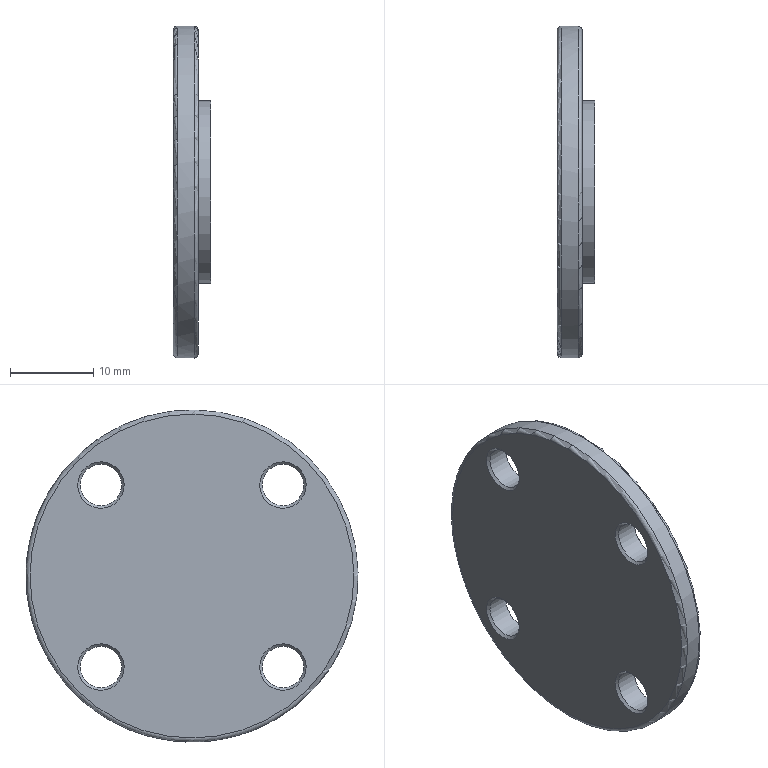Component | NX | UPPER_END_CAP_2 | 1 solid | 15 faces | box 4.5 x 40 x 40 mm | volume 4088 mm3 | cylinder 6 | cone 4 | plane 3 | torus 2 | commonest cylinder face diameters 5 x4 22 x1 40 x1
STEP:
#1=CARTESIAN_POINT('',(0.,0.,0.));
#2=DIRECTION('',(0.,0.,1.));
#3=DIRECTION('',(1.,0.,0.));
#4=AXIS2_PLACEMENT_3D('',#1,#2,#3);
#5=CARTESIAN_POINT('',(-135.,-29.778,26.278));
#6=VERTEX_POINT('',#5);
#7=CARTESIAN_POINT('',(-135.,-22.,18.5));
#8=DIRECTION('',(-1.,0.,0.));
#9=DIRECTION('',(0.,-0.7071,0.7071));
#10=AXIS2_PLACEMENT_3D('',#7,#8,#9);
#11=CIRCLE('',#10,11.);
#12=CARTESIAN_POINT('',(-135.,-22.,18.5));
#13=DIRECTION('',(1.,0.,0.));
#14=DIRECTION('',(0.,0.7071,-0.7071));
#15=AXIS2_PLACEMENT_3D('',#12,#13,#14);
#16=PLANE('',#15);
#17=CARTESIAN_POINT('',(-11.,-0.));
#18=CARTESIAN_POINT('',(-11.,19.053));
#19=CARTESIAN_POINT('',(5.5,9.526));
#20=CARTESIAN_POINT('',(22.,0.));
#21=CARTESIAN_POINT('',(5.5,-9.526));
#22=CARTESIAN_POINT('',(-11.,-19.053));
#23=CARTESIAN_POINT('',(-11.,-0.));
#24=(BOUNDED_CURVE()B_SPLINE_CURVE(2,(#17,#18,#19,#20,#21,#22,#23),.UNSPECIFIED.,.T.,.F.)B_SPLINE_CURVE_WITH_KNOTS((1,2,2,2,2,1),(-2.094,0.,2.094,4.189,6.283,8.378),.UNSPECIFIED.)CURVE()GEOMETRIC_REPRESENTATION_ITEM()RATIONAL_B_SPLINE_CURVE((1.,0.5,1.,0.5,1.,0.5,1.))REPRESENTATION_ITEM(''));
#25=(GEOMETRIC_REPRESENTATION_CONTEXT(2)PARAMETRIC_REPRESENTATION_CONTEXT()REPRESENTATION_CONTEXT('',''));
#26=DEFINITIONAL_REPRESENTATION('',(#24),#25);
#27=PCURVE('',#16,#26);
#28=CARTESIAN_POINT('',(-135.,-22.,18.5));
#29=DIRECTION('',(-1.,0.,0.));
#30=DIRECTION('',(0.,-0.7071,0.7071));
#31=AXIS2_PLACEMENT_3D('',#28,#29,#30);
#32=CYLINDRICAL_SURFACE('',#31,11.);
#33=CARTESIAN_POINT('',(0.,0.));
#34=DIRECTION('',(1.,0.));
#35=VECTOR('',#34,1.);
#36=LINE('',#33,#35);
#37=(GEOMETRIC_REPRESENTATION_CONTEXT(2)PARAMETRIC_REPRESENTATION_CONTEXT()REPRESENTATION_CONTEXT('',''));
#38=DEFINITIONAL_REPRESENTATION('',(#36),#37);
#39=PCURVE('',#32,#38);
#40=SURFACE_CURVE('',#11,(#27,#39),.PCURVE_S1.);
#41=EDGE_CURVE('',#6,#6,#40,.T.);
#42=ORIENTED_EDGE('',*,*,#41,.F.);
#43=EDGE_LOOP('',(#42));
#44=FACE_BOUND('',#43,.T.);
#45=ADVANCED_FACE('',(#44),#16,.T.);
#46=CARTESIAN_POINT('',(-136.5,-29.778,26.278));
#47=VERTEX_POINT('',#46);
#48=CARTESIAN_POINT('',(-136.5,-22.,18.5));
#49=DIRECTION('',(1.,0.,0.));
#50=DIRECTION('',(0.,-0.7071,0.7071));
#51=AXIS2_PLACEMENT_3D('',#48,#49,#50);
#52=CIRCLE('',#51,11.);
#53=CARTESIAN_POINT('',(6.283,1.5));
#54=DIRECTION('',(-1.,0.));
#55=VECTOR('',#54,1.);
#56=LINE('',#53,#55);
#57=(GEOMETRIC_REPRESENTATION_CONTEXT(2)PARAMETRIC_REPRESENTATION_CONTEXT()REPRESENTATION_CONTEXT('',''));
#58=DEFINITIONAL_REPRESENTATION('',(#56),#57);
#59=PCURVE('',#32,#58);
#60=CARTESIAN_POINT('',(-136.5,-22.,18.5));
#61=DIRECTION('',(1.,0.,0.));
#62=DIRECTION('',(0.,0.7071,-0.7071));
#63=AXIS2_PLACEMENT_3D('',#60,#61,#62);
#64=PLANE('',#63);
#65=CARTESIAN_POINT('',(0.,0.));
#66=DIRECTION('',(-1.,-0.));
#67=AXIS2_PLACEMENT_2D('',#65,#66);
#68=CIRCLE('',#67,11.);
#69=(GEOMETRIC_REPRESENTATION_CONTEXT(2)PARAMETRIC_REPRESENTATION_CONTEXT()REPRESENTATION_CONTEXT('',''));
#70=DEFINITIONAL_REPRESENTATION('',(#68),#69);
#71=PCURVE('',#64,#70);
#72=SURFACE_CURVE('',#52,(#59,#71),.PCURVE_S1.);
#73=EDGE_CURVE('',#47,#47,#72,.T.);
#74=ORIENTED_EDGE('',*,*,#73,.T.);
#75=CARTESIAN_POINT('',(-135.,-29.778,26.278));
#76=CARTESIAN_POINT('',(-136.5,-29.778,26.278));
#77=B_SPLINE_CURVE_WITH_KNOTS('',1,(#75,#76),.UNSPECIFIED.,.F.,.F.,(2,2),(0.,1.5),.PIECEWISE_BEZIER_KNOTS.);
#78=CARTESIAN_POINT('',(0.,0.));
#79=DIRECTION('',(0.,1.));
#80=VECTOR('',#79,1.);
#81=LINE('',#78,#80);
#82=(GEOMETRIC_REPRESENTATION_CONTEXT(2)PARAMETRIC_REPRESENTATION_CONTEXT()REPRESENTATION_CONTEXT('',''));
#83=DEFINITIONAL_REPRESENTATION('',(#81),#82);
#84=PCURVE('',#32,#83);
#85=CARTESIAN_POINT('',(6.283,0.));
#86=DIRECTION('',(0.,1.));
#87=VECTOR('',#86,1.);
#88=LINE('',#85,#87);
#89=(GEOMETRIC_REPRESENTATION_CONTEXT(2)PARAMETRIC_REPRESENTATION_CONTEXT()REPRESENTATION_CONTEXT('',''));
#90=DEFINITIONAL_REPRESENTATION('',(#88),#89);
#91=PCURVE('',#32,#90);
#92=SEAM_CURVE('',#77,(#84,#91),.PCURVE_S1.);
#93=EDGE_CURVE('',#6,#47,#92,.T.);
#94=ORIENTED_EDGE('',*,*,#93,.F.);
#95=ORIENTED_EDGE('',*,*,#41,.T.);
#96=ORIENTED_EDGE('',*,*,#93,.T.);
#97=EDGE_LOOP('',(#74,#94,#95,#96));
#98=FACE_BOUND('',#97,.T.);
#99=ADVANCED_FACE('',(#98),#32,.T.);
#100=CARTESIAN_POINT('',(-139.5,-13.02,9.52));
#101=VERTEX_POINT('',#100);
#102=CARTESIAN_POINT('',(-139.5,-11.04,7.54));
#103=DIRECTION('',(1.,0.,0.));
#104=DIRECTION('',(0.,-0.7071,0.7071));
#105=AXIS2_PLACEMENT_3D('',#102,#103,#104);
#106=CIRCLE('',#105,2.8);
#107=CARTESIAN_POINT('',(-139.5,-22.,18.5));
#108=DIRECTION('',(-1.,0.,0.));
#109=DIRECTION('',(0.,-0.7071,0.7071));
#110=AXIS2_PLACEMENT_3D('',#107,#108,#109);
#111=PLANE('',#110);
#112=CARTESIAN_POINT('',(-12.7,0.));
#113=CARTESIAN_POINT('',(-12.7,-4.85));
#114=CARTESIAN_POINT('',(-16.9,-2.425));
#115=CARTESIAN_POINT('',(-21.1,0.));
#116=CARTESIAN_POINT('',(-16.9,2.425));
#117=CARTESIAN_POINT('',(-12.7,4.85));
#118=CARTESIAN_POINT('',(-12.7,0.));
#119=(BOUNDED_CURVE()B_SPLINE_CURVE(2,(#112,#113,#114,#115,#116,#117,#118),.UNSPECIFIED.,.T.,.F.)B_SPLINE_CURVE_WITH_KNOTS((1,2,2,2,2,1),(-2.094,0.,2.094,4.189,6.283,8.378),.UNSPECIFIED.)CURVE()GEOMETRIC_REPRESENTATION_ITEM()RATIONAL_B_SPLINE_CURVE((1.,0.5,1.,0.5,1.,0.5,1.))REPRESENTATION_ITEM(''));
#120=(GEOMETRIC_REPRESENTATION_CONTEXT(2)PARAMETRIC_REPRESENTATION_CONTEXT()REPRESENTATION_CONTEXT('',''));
#121=DEFINITIONAL_REPRESENTATION('',(#119),#120);
#122=PCURVE('',#111,#121);
#123=CARTESIAN_POINT('',(-139.2,-11.04,7.54));
#124=DIRECTION('',(-1.,0.,0.));
#125=DIRECTION('',(0.,-0.7071,0.7071));
#126=AXIS2_PLACEMENT_3D('',#123,#124,#125);
#127=CONICAL_SURFACE('',#126,2.5,0.7854);
#128=CARTESIAN_POINT('',(6.283,0.3));
#129=DIRECTION('',(-1.,0.));
#130=VECTOR('',#129,1.);
#131=LINE('',#128,#130);
#132=(GEOMETRIC_REPRESENTATION_CONTEXT(2)PARAMETRIC_REPRESENTATION_CONTEXT()REPRESENTATION_CONTEXT('',''));
#133=DEFINITIONAL_REPRESENTATION('',(#131),#132);
#134=PCURVE('',#127,#133);
#135=SURFACE_CURVE('',#106,(#122,#134),.PCURVE_S1.);
#136=EDGE_CURVE('',#101,#101,#135,.T.);
#137=ORIENTED_EDGE('',*,*,#136,.T.);
#138=EDGE_LOOP('',(#137));
#139=FACE_BOUND('',#138,.T.);
#140=CARTESIAN_POINT('',(-139.5,-34.94,9.52));
#141=VERTEX_POINT('',#140);
#142=CARTESIAN_POINT('',(-139.5,-32.96,7.54));
#143=DIRECTION('',(1.,0.,0.));
#144=DIRECTION('',(0.,-0.7071,0.7071));
#145=AXIS2_PLACEMENT_3D('',#142,#143,#144);
#146=CIRCLE('',#145,2.8);
#147=CARTESIAN_POINT('',(2.8,-15.5));
#148=CARTESIAN_POINT('',(2.8,-20.35));
#149=CARTESIAN_POINT('',(-1.4,-17.925));
#150=CARTESIAN_POINT('',(-5.6,-15.5));
#151=CARTESIAN_POINT('',(-1.4,-13.075));
#152=CARTESIAN_POINT('',(2.8,-10.65));
#153=CARTESIAN_POINT('',(2.8,-15.5));
#154=(BOUNDED_CURVE()B_SPLINE_CURVE(2,(#147,#148,#149,#150,#151,#152,#153),.UNSPECIFIED.,.T.,.F.)B_SPLINE_CURVE_WITH_KNOTS((1,2,2,2,2,1),(-2.094,0.,2.094,4.189,6.283,8.378),.UNSPECIFIED.)CURVE()GEOMETRIC_REPRESENTATION_ITEM()RATIONAL_B_SPLINE_CURVE((1.,0.5,1.,0.5,1.,0.5,1.))REPRESENTATION_ITEM(''));
#155=(GEOMETRIC_REPRESENTATION_CONTEXT(2)PARAMETRIC_REPRESENTATION_CONTEXT()REPRESENTATION_CONTEXT('',''));
#156=DEFINITIONAL_REPRESENTATION('',(#154),#155);
#157=PCURVE('',#111,#156);
#158=CARTESIAN_POINT('',(-139.2,-32.96,7.54));
#159=DIRECTION('',(-1.,0.,0.));
#160=DIRECTION('',(0.,-0.7071,0.7071));
#161=AXIS2_PLACEMENT_3D('',#158,#159,#160);
#162=CONICAL_SURFACE('',#161,2.5,0.7854);
#163=CARTESIAN_POINT('',(6.283,0.3));
#164=DIRECTION('',(-1.,0.));
#165=VECTOR('',#164,1.);
#166=LINE('',#163,#165);
#167=(GEOMETRIC_REPRESENTATION_CONTEXT(2)PARAMETRIC_REPRESENTATION_CONTEXT()REPRESENTATION_CONTEXT('',''));
#168=DEFINITIONAL_REPRESENTATION('',(#166),#167);
#169=PCURVE('',#162,#168);
#170=SURFACE_CURVE('',#146,(#157,#169),.PCURVE_S1.);
#171=EDGE_CURVE('',#141,#141,#170,.T.);
#172=ORIENTED_EDGE('',*,*,#171,.T.);
#173=EDGE_LOOP('',(#172));
#174=FACE_BOUND('',#173,.T.);
#175=CARTESIAN_POINT('',(-139.5,-13.02,31.44));
#176=VERTEX_POINT('',#175);
#177=CARTESIAN_POINT('',(-139.5,-11.04,29.46));
#178=DIRECTION('',(1.,0.,0.));
#179=DIRECTION('',(0.,-0.7071,0.7071));
#180=AXIS2_PLACEMENT_3D('',#177,#178,#179);
#181=CIRCLE('',#180,2.8);
#182=CARTESIAN_POINT('',(2.8,15.5));
#183=CARTESIAN_POINT('',(2.8,10.65));
#184=CARTESIAN_POINT('',(-1.4,13.075));
#185=CARTESIAN_POINT('',(-5.6,15.5));
#186=CARTESIAN_POINT('',(-1.4,17.925));
#187=CARTESIAN_POINT('',(2.8,20.35));
#188=CARTESIAN_POINT('',(2.8,15.5));
#189=(BOUNDED_CURVE()B_SPLINE_CURVE(2,(#182,#183,#184,#185,#186,#187,#188),.UNSPECIFIED.,.T.,.F.)B_SPLINE_CURVE_WITH_KNOTS((1,2,2,2,2,1),(-2.094,0.,2.094,4.189,6.283,8.378),.UNSPECIFIED.)CURVE()GEOMETRIC_REPRESENTATION_ITEM()RATIONAL_B_SPLINE_CURVE((1.,0.5,1.,0.5,1.,0.5,1.))REPRESENTATION_ITEM(''));
#190=(GEOMETRIC_REPRESENTATION_CONTEXT(2)PARAMETRIC_REPRESENTATION_CONTEXT()REPRESENTATION_CONTEXT('',''));
#191=DEFINITIONAL_REPRESENTATION('',(#189),#190);
#192=PCURVE('',#111,#191);
#193=CARTESIAN_POINT('',(-139.2,-11.04,29.46));
#194=DIRECTION('',(-1.,0.,0.));
#195=DIRECTION('',(0.,-0.7071,0.7071));
#196=AXIS2_PLACEMENT_3D('',#193,#194,#195);
#197=CONICAL_SURFACE('',#196,2.5,0.7854);
#198=CARTESIAN_POINT('',(6.283,0.3));
#199=DIRECTION('',(-1.,0.));
#200=VECTOR('',#199,1.);
#201=LINE('',#198,#200);
#202=(GEOMETRIC_REPRESENTATION_CONTEXT(2)PARAMETRIC_REPRESENTATION_CONTEXT()REPRESENTATION_CONTEXT('',''));
#203=DEFINITIONAL_REPRESENTATION('',(#201),#202);
#204=PCURVE('',#197,#203);
#205=SURFACE_CURVE('',#181,(#192,#204),.PCURVE_S1.);
#206=EDGE_CURVE('',#176,#176,#205,.T.);
#207=ORIENTED_EDGE('',*,*,#206,.T.);
#208=EDGE_LOOP('',(#207));
#209=FACE_BOUND('',#208,.T.);
#210=CARTESIAN_POINT('',(-139.5,-34.94,31.44));
#211=VERTEX_POINT('',#210);
#212=CARTESIAN_POINT('',(-139.5,-32.96,29.46));
#213=DIRECTION('',(1.,0.,0.));
#214=DIRECTION('',(0.,-0.7071,0.7071));
#215=AXIS2_PLACEMENT_3D('',#212,#213,#214);
#216=CIRCLE('',#215,2.8);
#217=CARTESIAN_POINT('',(18.3,0.));
#218=CARTESIAN_POINT('',(18.3,-4.85));
#219=CARTESIAN_POINT('',(14.1,-2.425));
#220=CARTESIAN_POINT('',(9.9,0.));
#221=CARTESIAN_POINT('',(14.1,2.425));
#222=CARTESIAN_POINT('',(18.3,4.85));
#223=CARTESIAN_POINT('',(18.3,0.));
#224=(BOUNDED_CURVE()B_SPLINE_CURVE(2,(#217,#218,#219,#220,#221,#222,#223),.UNSPECIFIED.,.T.,.F.)B_SPLINE_CURVE_WITH_KNOTS((1,2,2,2,2,1),(-2.094,0.,2.094,4.189,6.283,8.378),.UNSPECIFIED.)CURVE()GEOMETRIC_REPRESENTATION_ITEM()RATIONAL_B_SPLINE_CURVE((1.,0.5,1.,0.5,1.,0.5,1.))REPRESENTATION_ITEM(''));
#225=(GEOMETRIC_REPRESENTATION_CONTEXT(2)PARAMETRIC_REPRESENTATION_CONTEXT()REPRESENTATION_CONTEXT('',''));
#226=DEFINITIONAL_REPRESENTATION('',(#224),#225);
#227=PCURVE('',#111,#226);
#228=CARTESIAN_POINT('',(-139.2,-32.96,29.46));
#229=DIRECTION('',(-1.,0.,0.));
#230=DIRECTION('',(0.,-0.7071,0.7071));
#231=AXIS2_PLACEMENT_3D('',#228,#229,#230);
#232=CONICAL_SURFACE('',#231,2.5,0.7854);
#233=CARTESIAN_POINT('',(6.283,0.3));
#234=DIRECTION('',(-1.,0.));
#235=VECTOR('',#234,1.);
#236=LINE('',#233,#235);
#237=(GEOMETRIC_REPRESENTATION_CONTEXT(2)PARAMETRIC_REPRESENTATION_CONTEXT()REPRESENTATION_CONTEXT('',''));
#238=DEFINITIONAL_REPRESENTATION('',(#236),#237);
#239=PCURVE('',#232,#238);
#240=SURFACE_CURVE('',#216,(#227,#239),.PCURVE_S1.);
#241=EDGE_CURVE('',#211,#211,#240,.T.);
#242=ORIENTED_EDGE('',*,*,#241,.T.);
#243=EDGE_LOOP('',(#242));
#244=FACE_BOUND('',#243,.T.);
#245=CARTESIAN_POINT('',(-139.5,-35.789,32.289));
#246=VERTEX_POINT('',#245);
#247=CARTESIAN_POINT('',(-139.5,-22.,18.5));
#248=DIRECTION('',(-1.,0.,0.));
#249=DIRECTION('',(0.,-0.7071,0.7071));
#250=AXIS2_PLACEMENT_3D('',#247,#248,#249);
#251=CIRCLE('',#250,19.5);
#252=CARTESIAN_POINT('',(0.,0.));
#253=DIRECTION('',(1.,0.));
#254=AXIS2_PLACEMENT_2D('',#252,#253);
#255=CIRCLE('',#254,19.5);
#256=(GEOMETRIC_REPRESENTATION_CONTEXT(2)PARAMETRIC_REPRESENTATION_CONTEXT()REPRESENTATION_CONTEXT('',''));
#257=DEFINITIONAL_REPRESENTATION('',(#255),#256);
#258=PCURVE('',#111,#257);
#259=CARTESIAN_POINT('',(-139.,-22.,18.5));
#260=DIRECTION('',(-1.,0.,0.));
#261=DIRECTION('',(0.,-0.7071,0.7071));
#262=AXIS2_PLACEMENT_3D('',#259,#260,#261);
#263=TOROIDAL_SURFACE('',#262,19.5,0.5);
#264=CARTESIAN_POINT('',(0.,7.854));
#265=DIRECTION('',(1.,0.));
#266=VECTOR('',#265,1.);
#267=LINE('',#264,#266);
#268=(GEOMETRIC_REPRESENTATION_CONTEXT(2)PARAMETRIC_REPRESENTATION_CONTEXT()REPRESENTATION_CONTEXT('',''));
#269=DEFINITIONAL_REPRESENTATION('',(#267),#268);
#270=PCURVE('',#263,#269);
#271=SURFACE_CURVE('',#251,(#258,#270),.PCURVE_S1.);
#272=EDGE_CURVE('',#246,#246,#271,.T.);
#273=ORIENTED_EDGE('',*,*,#272,.T.);
#274=EDGE_LOOP('',(#273));
#275=FACE_BOUND('',#274,.T.);
#276=ADVANCED_FACE('',(#139,#174,#209,#244,#275),#111,.T.);
#277=CARTESIAN_POINT('',(-136.5,-31.192,27.692));
#278=VERTEX_POINT('',#277);
#279=CARTESIAN_POINT('',(-136.5,-34.728,31.228));
#280=VERTEX_POINT('',#279);
#281=CARTESIAN_POINT('',(-136.5,-32.96,29.46));
#282=DIRECTION('',(1.,0.,0.));
#283=DIRECTION('',(0.,0.7071,-0.7071));
#284=AXIS2_PLACEMENT_3D('',#281,#282,#283);
#285=CIRCLE('',#284,2.5);
#286=CARTESIAN_POINT('',(-15.5,0.));
#287=DIRECTION('',(1.,0.));
#288=AXIS2_PLACEMENT_2D('',#286,#287);
#289=CIRCLE('',#288,2.5);
#290=(GEOMETRIC_REPRESENTATION_CONTEXT(2)PARAMETRIC_REPRESENTATION_CONTEXT()REPRESENTATION_CONTEXT('',''));
#291=DEFINITIONAL_REPRESENTATION('',(#289),#290);
#292=PCURVE('',#64,#291);
#293=CARTESIAN_POINT('',(-119.5,-32.96,29.46));
#294=DIRECTION('',(-1.,0.,0.));
#295=DIRECTION('',(0.,-0.7071,0.7071));
#296=AXIS2_PLACEMENT_3D('',#293,#294,#295);
#297=CYLINDRICAL_SURFACE('',#296,2.5);
#298=CARTESIAN_POINT('',(3.142,17.));
#299=DIRECTION('',(-1.,0.));
#300=VECTOR('',#299,1.);
#301=LINE('',#298,#300);
#302=(GEOMETRIC_REPRESENTATION_CONTEXT(2)PARAMETRIC_REPRESENTATION_CONTEXT()REPRESENTATION_CONTEXT('',''));
#303=DEFINITIONAL_REPRESENTATION('',(#301),#302);
#304=PCURVE('',#297,#303);
#305=SURFACE_CURVE('',#285,(#292,#304),.PCURVE_S1.);
#306=EDGE_CURVE('',#278,#280,#305,.T.);
#307=ORIENTED_EDGE('',*,*,#306,.F.);
#308=CARTESIAN_POINT('',(-136.5,-32.96,29.46));
#309=DIRECTION('',(1.,0.,0.));
#310=DIRECTION('',(0.,0.7071,-0.7071));
#311=AXIS2_PLACEMENT_3D('',#308,#309,#310);
#312=CIRCLE('',#311,2.5);
#313=CARTESIAN_POINT('',(-15.5,0.));
#314=DIRECTION('',(1.,0.));
#315=AXIS2_PLACEMENT_2D('',#313,#314);
#316=CIRCLE('',#315,2.5);
#317=(GEOMETRIC_REPRESENTATION_CONTEXT(2)PARAMETRIC_REPRESENTATION_CONTEXT()REPRESENTATION_CONTEXT('',''));
#318=DEFINITIONAL_REPRESENTATION('',(#316),#317);
#319=PCURVE('',#64,#318);
#320=CARTESIAN_POINT('',(9.425,17.));
#321=DIRECTION('',(-1.,0.));
#322=VECTOR('',#321,1.);
#323=LINE('',#320,#322);
#324=(GEOMETRIC_REPRESENTATION_CONTEXT(2)PARAMETRIC_REPRESENTATION_CONTEXT()REPRESENTATION_CONTEXT('',''));
#325=DEFINITIONAL_REPRESENTATION('',(#323),#324);
#326=PCURVE('',#297,#325);
#327=SURFACE_CURVE('',#312,(#319,#326),.PCURVE_S1.);
#328=EDGE_CURVE('',#280,#278,#327,.T.);
#329=ORIENTED_EDGE('',*,*,#328,.F.);
#330=EDGE_LOOP('',(#307,#329));
#331=FACE_BOUND('',#330,.T.);
#332=CARTESIAN_POINT('',(-136.5,-9.272,27.692));
#333=VERTEX_POINT('',#332);
#334=CARTESIAN_POINT('',(-136.5,-12.808,31.228));
#335=VERTEX_POINT('',#334);
#336=CARTESIAN_POINT('',(-136.5,-11.04,29.46));
#337=DIRECTION('',(1.,0.,0.));
#338=DIRECTION('',(0.,0.7071,-0.7071));
#339=AXIS2_PLACEMENT_3D('',#336,#337,#338);
#340=CIRCLE('',#339,2.5);
#341=CARTESIAN_POINT('',(-0.,15.5));
#342=DIRECTION('',(1.,0.));
#343=AXIS2_PLACEMENT_2D('',#341,#342);
#344=CIRCLE('',#343,2.5);
#345=(GEOMETRIC_REPRESENTATION_CONTEXT(2)PARAMETRIC_REPRESENTATION_CONTEXT()REPRESENTATION_CONTEXT('',''));
#346=DEFINITIONAL_REPRESENTATION('',(#344),#345);
#347=PCURVE('',#64,#346);
#348=CARTESIAN_POINT('',(-119.5,-11.04,29.46));
#349=DIRECTION('',(-1.,0.,0.));
#350=DIRECTION('',(0.,-0.7071,0.7071));
#351=AXIS2_PLACEMENT_3D('',#348,#349,#350);
#352=CYLINDRICAL_SURFACE('',#351,2.5);
#353=CARTESIAN_POINT('',(3.142,17.));
#354=DIRECTION('',(-1.,0.));
#355=VECTOR('',#354,1.);
#356=LINE('',#353,#355);
#357=(GEOMETRIC_REPRESENTATION_CONTEXT(2)PARAMETRIC_REPRESENTATION_CONTEXT()REPRESENTATION_CONTEXT('',''));
#358=DEFINITIONAL_REPRESENTATION('',(#356),#357);
#359=PCURVE('',#352,#358);
#360=SURFACE_CURVE('',#340,(#347,#359),.PCURVE_S1.);
#361=EDGE_CURVE('',#333,#335,#360,.T.);
#362=ORIENTED_EDGE('',*,*,#361,.F.);
#363=CARTESIAN_POINT('',(-136.5,-11.04,29.46));
#364=DIRECTION('',(1.,0.,0.));
#365=DIRECTION('',(0.,0.7071,-0.7071));
#366=AXIS2_PLACEMENT_3D('',#363,#364,#365);
#367=CIRCLE('',#366,2.5);
#368=CARTESIAN_POINT('',(-0.,15.5));
#369=DIRECTION('',(1.,0.));
#370=AXIS2_PLACEMENT_2D('',#368,#369);
#371=CIRCLE('',#370,2.5);
#372=(GEOMETRIC_REPRESENTATION_CONTEXT(2)PARAMETRIC_REPRESENTATION_CONTEXT()REPRESENTATION_CONTEXT('',''));
#373=DEFINITIONAL_REPRESENTATION('',(#371),#372);
#374=PCURVE('',#64,#373);
#375=CARTESIAN_POINT('',(9.425,17.));
#376=DIRECTION('',(-1.,0.));
#377=VECTOR('',#376,1.);
#378=LINE('',#375,#377);
#379=(GEOMETRIC_REPRESENTATION_CONTEXT(2)PARAMETRIC_REPRESENTATION_CONTEXT()REPRESENTATION_CONTEXT('',''));
#380=DEFINITIONAL_REPRESENTATION('',(#378),#379);
#381=PCURVE('',#352,#380);
#382=SURFACE_CURVE('',#367,(#374,#381),.PCURVE_S1.);
#383=EDGE_CURVE('',#335,#333,#382,.T.);
#384=ORIENTED_EDGE('',*,*,#383,.F.);
#385=EDGE_LOOP('',(#362,#384));
#386=FACE_BOUND('',#385,.T.);
#387=CARTESIAN_POINT('',(-136.5,-31.192,5.772));
#388=VERTEX_POINT('',#387);
#389=CARTESIAN_POINT('',(-136.5,-34.728,9.308));
#390=VERTEX_POINT('',#389);
#391=CARTESIAN_POINT('',(-136.5,-32.96,7.54));
#392=DIRECTION('',(1.,0.,0.));
#393=DIRECTION('',(0.,0.7071,-0.7071));
#394=AXIS2_PLACEMENT_3D('',#391,#392,#393);
#395=CIRCLE('',#394,2.5);
#396=CARTESIAN_POINT('',(-0.,-15.5));
#397=DIRECTION('',(1.,0.));
#398=AXIS2_PLACEMENT_2D('',#396,#397);
#399=CIRCLE('',#398,2.5);
#400=(GEOMETRIC_REPRESENTATION_CONTEXT(2)PARAMETRIC_REPRESENTATION_CONTEXT()REPRESENTATION_CONTEXT('',''));
#401=DEFINITIONAL_REPRESENTATION('',(#399),#400);
#402=PCURVE('',#64,#401);
#403=CARTESIAN_POINT('',(-119.5,-32.96,7.54));
#404=DIRECTION('',(-1.,0.,0.));
#405=DIRECTION('',(0.,-0.7071,0.7071));
#406=AXIS2_PLACEMENT_3D('',#403,#404,#405);
#407=CYLINDRICAL_SURFACE('',#406,2.5);
#408=CARTESIAN_POINT('',(3.142,17.));
#409=DIRECTION('',(-1.,0.));
#410=VECTOR('',#409,1.);
#411=LINE('',#408,#410);
#412=(GEOMETRIC_REPRESENTATION_CONTEXT(2)PARAMETRIC_REPRESENTATION_CONTEXT()REPRESENTATION_CONTEXT('',''));
#413=DEFINITIONAL_REPRESENTATION('',(#411),#412);
#414=PCURVE('',#407,#413);
#415=SURFACE_CURVE('',#395,(#402,#414),.PCURVE_S1.);
#416=EDGE_CURVE('',#388,#390,#415,.T.);
#417=ORIENTED_EDGE('',*,*,#416,.F.);
#418=CARTESIAN_POINT('',(-136.5,-32.96,7.54));
#419=DIRECTION('',(1.,0.,0.));
#420=DIRECTION('',(0.,0.7071,-0.7071));
#421=AXIS2_PLACEMENT_3D('',#418,#419,#420);
#422=CIRCLE('',#421,2.5);
#423=CARTESIAN_POINT('',(-0.,-15.5));
#424=DIRECTION('',(1.,0.));
#425=AXIS2_PLACEMENT_2D('',#423,#424);
#426=CIRCLE('',#425,2.5);
#427=(GEOMETRIC_REPRESENTATION_CONTEXT(2)PARAMETRIC_REPRESENTATION_CONTEXT()REPRESENTATION_CONTEXT('',''));
#428=DEFINITIONAL_REPRESENTATION('',(#426),#427);
#429=PCURVE('',#64,#428);
#430=CARTESIAN_POINT('',(9.425,17.));
#431=DIRECTION('',(-1.,0.));
#432=VECTOR('',#431,1.);
#433=LINE('',#430,#432);
#434=(GEOMETRIC_REPRESENTATION_CONTEXT(2)PARAMETRIC_REPRESENTATION_CONTEXT()REPRESENTATION_CONTEXT('',''));
#435=DEFINITIONAL_REPRESENTATION('',(#433),#434);
#436=PCURVE('',#407,#435);
#437=SURFACE_CURVE('',#422,(#429,#436),.PCURVE_S1.);
#438=EDGE_CURVE('',#390,#388,#437,.T.);
#439=ORIENTED_EDGE('',*,*,#438,.F.);
#440=EDGE_LOOP('',(#417,#439));
#441=FACE_BOUND('',#440,.T.);
#442=CARTESIAN_POINT('',(-136.5,-9.272,5.772));
#443=VERTEX_POINT('',#442);
#444=CARTESIAN_POINT('',(-136.5,-12.808,9.308));
#445=VERTEX_POINT('',#444);
#446=CARTESIAN_POINT('',(-136.5,-11.04,7.54));
#447=DIRECTION('',(1.,0.,0.));
#448=DIRECTION('',(0.,0.7071,-0.7071));
#449=AXIS2_PLACEMENT_3D('',#446,#447,#448);
#450=CIRCLE('',#449,2.5);
#451=CARTESIAN_POINT('',(15.5,0.));
#452=DIRECTION('',(1.,0.));
#453=AXIS2_PLACEMENT_2D('',#451,#452);
#454=CIRCLE('',#453,2.5);
#455=(GEOMETRIC_REPRESENTATION_CONTEXT(2)PARAMETRIC_REPRESENTATION_CONTEXT()REPRESENTATION_CONTEXT('',''));
#456=DEFINITIONAL_REPRESENTATION('',(#454),#455);
#457=PCURVE('',#64,#456);
#458=CARTESIAN_POINT('',(-119.5,-11.04,7.54));
#459=DIRECTION('',(-1.,0.,0.));
#460=DIRECTION('',(0.,-0.7071,0.7071));
#461=AXIS2_PLACEMENT_3D('',#458,#459,#460);
#462=CYLINDRICAL_SURFACE('',#461,2.5);
#463=CARTESIAN_POINT('',(3.142,17.));
#464=DIRECTION('',(-1.,0.));
#465=VECTOR('',#464,1.);
#466=LINE('',#463,#465);
#467=(GEOMETRIC_REPRESENTATION_CONTEXT(2)PARAMETRIC_REPRESENTATION_CONTEXT()REPRESENTATION_CONTEXT('',''));
#468=DEFINITIONAL_REPRESENTATION('',(#466),#467);
#469=PCURVE('',#462,#468);
#470=SURFACE_CURVE('',#450,(#457,#469),.PCURVE_S1.);
#471=EDGE_CURVE('',#443,#445,#470,.T.);
#472=ORIENTED_EDGE('',*,*,#471,.F.);
#473=CARTESIAN_POINT('',(-136.5,-11.04,7.54));
#474=DIRECTION('',(1.,0.,0.));
#475=DIRECTION('',(0.,0.7071,-0.7071));
#476=AXIS2_PLACEMENT_3D('',#473,#474,#475);
#477=CIRCLE('',#476,2.5);
#478=CARTESIAN_POINT('',(15.5,0.));
#479=DIRECTION('',(1.,0.));
#480=AXIS2_PLACEMENT_2D('',#478,#479);
#481=CIRCLE('',#480,2.5);
#482=(GEOMETRIC_REPRESENTATION_CONTEXT(2)PARAMETRIC_REPRESENTATION_CONTEXT()REPRESENTATION_CONTEXT('',''));
#483=DEFINITIONAL_REPRESENTATION('',(#481),#482);
#484=PCURVE('',#64,#483);
#485=CARTESIAN_POINT('',(9.425,17.));
#486=DIRECTION('',(-1.,0.));
#487=VECTOR('',#486,1.);
#488=LINE('',#485,#487);
#489=(GEOMETRIC_REPRESENTATION_CONTEXT(2)PARAMETRIC_REPRESENTATION_CONTEXT()REPRESENTATION_CONTEXT('',''));
#490=DEFINITIONAL_REPRESENTATION('',(#488),#489);
#491=PCURVE('',#462,#490);
#492=SURFACE_CURVE('',#477,(#484,#491),.PCURVE_S1.);
#493=EDGE_CURVE('',#445,#443,#492,.T.);
#494=ORIENTED_EDGE('',*,*,#493,.F.);
#495=EDGE_LOOP('',(#472,#494));
#496=FACE_BOUND('',#495,.T.);
#497=CARTESIAN_POINT('',(-136.5,-8.211,4.711));
#498=VERTEX_POINT('',#497);
#499=CARTESIAN_POINT('',(-136.5,-22.,18.5));
#500=DIRECTION('',(1.,0.,0.));
#501=DIRECTION('',(0.,0.7071,-0.7071));
#502=AXIS2_PLACEMENT_3D('',#499,#500,#501);
#503=CIRCLE('',#502,19.5);
#504=CARTESIAN_POINT('',(0.,0.));
#505=DIRECTION('',(1.,0.));
#506=AXIS2_PLACEMENT_2D('',#504,#505);
#507=CIRCLE('',#506,19.5);
#508=(GEOMETRIC_REPRESENTATION_CONTEXT(2)PARAMETRIC_REPRESENTATION_CONTEXT()REPRESENTATION_CONTEXT('',''));
#509=DEFINITIONAL_REPRESENTATION('',(#507),#508);
#510=PCURVE('',#64,#509);
#511=CARTESIAN_POINT('',(-137.,-22.,18.5));
#512=DIRECTION('',(1.,0.,0.));
#513=DIRECTION('',(0.,0.7071,-0.7071));
#514=AXIS2_PLACEMENT_3D('',#511,#512,#513);
#515=TOROIDAL_SURFACE('',#514,19.5,0.5);
#516=CARTESIAN_POINT('',(0.,7.854));
#517=DIRECTION('',(1.,0.));
#518=VECTOR('',#517,1.);
#519=LINE('',#516,#518);
#520=(GEOMETRIC_REPRESENTATION_CONTEXT(2)PARAMETRIC_REPRESENTATION_CONTEXT()REPRESENTATION_CONTEXT('',''));
#521=DEFINITIONAL_REPRESENTATION('',(#519),#520);
#522=PCURVE('',#515,#521);
#523=SURFACE_CURVE('',#503,(#510,#522),.PCURVE_S1.);
#524=EDGE_CURVE('',#498,#498,#523,.T.);
#525=ORIENTED_EDGE('',*,*,#524,.T.);
#526=EDGE_LOOP('',(#525));
#527=FACE_BOUND('',#526,.T.);
#528=ORIENTED_EDGE('',*,*,#73,.F.);
#529=EDGE_LOOP('',(#528));
#530=FACE_BOUND('',#529,.T.);
#531=ADVANCED_FACE('',(#331,#386,#441,#496,#527,#530),#64,.T.);
#532=CARTESIAN_POINT('',(-137.,-7.858,4.358));
#533=VERTEX_POINT('',#532);
#534=CARTESIAN_POINT('',(-137.,-36.142,32.642));
#535=VERTEX_POINT('',#534);
#536=CARTESIAN_POINT('',(-137.,-22.,18.5));
#537=DIRECTION('',(-1.,0.,0.));
#538=DIRECTION('',(0.,0.7071,-0.7071));
#539=AXIS2_PLACEMENT_3D('',#536,#537,#538);
#540=CIRCLE('',#539,20.);
#541=CARTESIAN_POINT('',(-136.5,-22.,18.5));
#542=DIRECTION('',(-1.,0.,0.));
#543=DIRECTION('',(0.,-0.7071,0.7071));
#544=AXIS2_PLACEMENT_3D('',#541,#542,#543);
#545=CYLINDRICAL_SURFACE('',#544,20.);
#546=CARTESIAN_POINT('',(3.142,0.5));
#547=DIRECTION('',(1.,0.));
#548=VECTOR('',#547,1.);
#549=LINE('',#546,#548);
#550=(GEOMETRIC_REPRESENTATION_CONTEXT(2)PARAMETRIC_REPRESENTATION_CONTEXT()REPRESENTATION_CONTEXT('',''));
#551=DEFINITIONAL_REPRESENTATION('',(#549),#550);
#552=PCURVE('',#545,#551);
#553=CARTESIAN_POINT('',(6.283,6.283));
#554=DIRECTION('',(-1.,0.));
#555=VECTOR('',#554,1.);
#556=LINE('',#553,#555);
#557=(GEOMETRIC_REPRESENTATION_CONTEXT(2)PARAMETRIC_REPRESENTATION_CONTEXT()REPRESENTATION_CONTEXT('',''));
#558=DEFINITIONAL_REPRESENTATION('',(#556),#557);
#559=PCURVE('',#515,#558);
#560=SURFACE_CURVE('',#540,(#552,#559),.PCURVE_S1.);
#561=EDGE_CURVE('',#533,#535,#560,.T.);
#562=ORIENTED_EDGE('',*,*,#561,.T.);
#563=CARTESIAN_POINT('',(-139.,-36.142,32.642));
#564=VERTEX_POINT('',#563);
#565=CARTESIAN_POINT('',(-137.,-36.142,32.642));
#566=CARTESIAN_POINT('',(-139.,-36.142,32.642));
#567=B_SPLINE_CURVE_WITH_KNOTS('',1,(#565,#566),.UNSPECIFIED.,.F.,.F.,(2,2),(0.5,2.5),.PIECEWISE_BEZIER_KNOTS.);
#568=CARTESIAN_POINT('',(6.283,0.));
#569=DIRECTION('',(0.,1.));
#570=VECTOR('',#569,1.);
#571=LINE('',#568,#570);
#572=(GEOMETRIC_REPRESENTATION_CONTEXT(2)PARAMETRIC_REPRESENTATION_CONTEXT()REPRESENTATION_CONTEXT('',''));
#573=DEFINITIONAL_REPRESENTATION('',(#571),#572);
#574=PCURVE('',#545,#573);
#575=CARTESIAN_POINT('',(0.,0.));
#576=DIRECTION('',(0.,1.));
#577=VECTOR('',#576,1.);
#578=LINE('',#575,#577);
#579=(GEOMETRIC_REPRESENTATION_CONTEXT(2)PARAMETRIC_REPRESENTATION_CONTEXT()REPRESENTATION_CONTEXT('',''));
#580=DEFINITIONAL_REPRESENTATION('',(#578),#579);
#581=PCURVE('',#545,#580);
#582=SEAM_CURVE('',#567,(#574,#581),.PCURVE_S1.);
#583=EDGE_CURVE('',#535,#564,#582,.T.);
#584=ORIENTED_EDGE('',*,*,#583,.T.);
#585=CARTESIAN_POINT('',(-139.,-22.,18.5));
#586=DIRECTION('',(1.,0.,0.));
#587=DIRECTION('',(0.,-0.7071,0.7071));
#588=AXIS2_PLACEMENT_3D('',#585,#586,#587);
#589=CIRCLE('',#588,20.);
#590=CARTESIAN_POINT('',(6.283,2.5));
#591=DIRECTION('',(-1.,0.));
#592=VECTOR('',#591,1.);
#593=LINE('',#590,#592);
#594=(GEOMETRIC_REPRESENTATION_CONTEXT(2)PARAMETRIC_REPRESENTATION_CONTEXT()REPRESENTATION_CONTEXT('',''));
#595=DEFINITIONAL_REPRESENTATION('',(#593),#594);
#596=PCURVE('',#545,#595);
#597=CARTESIAN_POINT('',(6.283,6.283));
#598=DIRECTION('',(-1.,0.));
#599=VECTOR('',#598,1.);
#600=LINE('',#597,#599);
#601=(GEOMETRIC_REPRESENTATION_CONTEXT(2)PARAMETRIC_REPRESENTATION_CONTEXT()REPRESENTATION_CONTEXT('',''));
#602=DEFINITIONAL_REPRESENTATION('',(#600),#601);
#603=PCURVE('',#263,#602);
#604=SURFACE_CURVE('',#589,(#596,#603),.PCURVE_S1.);
#605=EDGE_CURVE('',#564,#564,#604,.T.);
#606=ORIENTED_EDGE('',*,*,#605,.T.);
#607=ORIENTED_EDGE('',*,*,#583,.F.);
#608=CARTESIAN_POINT('',(-137.,-22.,18.5));
#609=DIRECTION('',(-1.,0.,0.));
#610=DIRECTION('',(0.,0.7071,-0.7071));
#611=AXIS2_PLACEMENT_3D('',#608,#609,#610);
#612=CIRCLE('',#611,20.);
#613=CARTESIAN_POINT('',(-3.142,0.5));
#614=DIRECTION('',(1.,0.));
#615=VECTOR('',#614,1.);
#616=LINE('',#613,#615);
#617=(GEOMETRIC_REPRESENTATION_CONTEXT(2)PARAMETRIC_REPRESENTATION_CONTEXT()REPRESENTATION_CONTEXT('',''));
#618=DEFINITIONAL_REPRESENTATION('',(#616),#617);
#619=PCURVE('',#545,#618);
#620=CARTESIAN_POINT('',(6.283,6.283));
#621=DIRECTION('',(-1.,0.));
#622=VECTOR('',#621,1.);
#623=LINE('',#620,#622);
#624=(GEOMETRIC_REPRESENTATION_CONTEXT(2)PARAMETRIC_REPRESENTATION_CONTEXT()REPRESENTATION_CONTEXT('',''));
#625=DEFINITIONAL_REPRESENTATION('',(#623),#624);
#626=PCURVE('',#515,#625);
#627=SURFACE_CURVE('',#612,(#619,#626),.PCURVE_S1.);
#628=EDGE_CURVE('',#535,#533,#627,.T.);
#629=ORIENTED_EDGE('',*,*,#628,.T.);
#630=EDGE_LOOP('',(#562,#584,#606,#607,#629));
#631=FACE_BOUND('',#630,.T.);
#632=ADVANCED_FACE('',(#631),#545,.T.);
#633=ORIENTED_EDGE('',*,*,#524,.F.);
#634=CARTESIAN_POINT('',(-137.,-7.858,4.358));
#635=CARTESIAN_POINT('',(-136.866,-7.858,4.358));
#636=CARTESIAN_POINT('',(-136.736,-7.888,4.388));
#637=CARTESIAN_POINT('',(-136.624,-7.946,4.446));
#638=CARTESIAN_POINT('',(-136.543,-8.025,4.525));
#639=CARTESIAN_POINT('',(-136.5,-8.117,4.617));
#640=CARTESIAN_POINT('',(-136.5,-8.211,4.711));
#641=(BOUNDED_CURVE()B_SPLINE_CURVE(6,(#634,#635,#636,#637,#638,#639,#640),.UNSPECIFIED.,.F.,.F.)B_SPLINE_CURVE_WITH_KNOTS((7,7),(0.,1.571),.PIECEWISE_BEZIER_KNOTS.)CURVE()GEOMETRIC_REPRESENTATION_ITEM()RATIONAL_B_SPLINE_CURVE((1.031,1.01,0.9979,0.994,0.9979,1.01,1.031))REPRESENTATION_ITEM(''));
#642=CARTESIAN_POINT('',(0.,6.283));
#643=DIRECTION('',(0.,1.));
#644=VECTOR('',#643,1.);
#645=LINE('',#642,#644);
#646=(GEOMETRIC_REPRESENTATION_CONTEXT(2)PARAMETRIC_REPRESENTATION_CONTEXT()REPRESENTATION_CONTEXT('',''));
#647=DEFINITIONAL_REPRESENTATION('',(#645),#646);
#648=PCURVE('',#515,#647);
#649=CARTESIAN_POINT('',(6.283,6.283));
#650=DIRECTION('',(0.,1.));
#651=VECTOR('',#650,1.);
#652=LINE('',#649,#651);
#653=(GEOMETRIC_REPRESENTATION_CONTEXT(2)PARAMETRIC_REPRESENTATION_CONTEXT()REPRESENTATION_CONTEXT('',''));
#654=DEFINITIONAL_REPRESENTATION('',(#652),#653);
#655=PCURVE('',#515,#654);
#656=SEAM_CURVE('',#641,(#648,#655),.PCURVE_S1.);
#657=EDGE_CURVE('',#533,#498,#656,.T.);
#658=ORIENTED_EDGE('',*,*,#657,.F.);
#659=ORIENTED_EDGE('',*,*,#628,.F.);
#660=ORIENTED_EDGE('',*,*,#561,.F.);
#661=ORIENTED_EDGE('',*,*,#657,.T.);
#662=EDGE_LOOP('',(#633,#658,#659,#660,#661));
#663=FACE_BOUND('',#662,.T.);
#664=ADVANCED_FACE('',(#663),#515,.T.);
#665=ORIENTED_EDGE('',*,*,#605,.F.);
#666=CARTESIAN_POINT('',(-139.,-36.142,32.642));
#667=CARTESIAN_POINT('',(-139.134,-36.142,32.642));
#668=CARTESIAN_POINT('',(-139.264,-36.112,32.612));
#669=CARTESIAN_POINT('',(-139.376,-36.054,32.554));
#670=CARTESIAN_POINT('',(-139.457,-35.975,32.475));
#671=CARTESIAN_POINT('',(-139.5,-35.883,32.383));
#672=CARTESIAN_POINT('',(-139.5,-35.789,32.289));
#673=(BOUNDED_CURVE()B_SPLINE_CURVE(6,(#666,#667,#668,#669,#670,#671,#672),.UNSPECIFIED.,.F.,.F.)B_SPLINE_CURVE_WITH_KNOTS((7,7),(0.,1.571),.PIECEWISE_BEZIER_KNOTS.)CURVE()GEOMETRIC_REPRESENTATION_ITEM()RATIONAL_B_SPLINE_CURVE((1.031,1.01,0.9979,0.994,0.9979,1.01,1.031))REPRESENTATION_ITEM(''));
#674=CARTESIAN_POINT('',(6.283,6.283));
#675=DIRECTION('',(0.,1.));
#676=VECTOR('',#675,1.);
#677=LINE('',#674,#676);
#678=(GEOMETRIC_REPRESENTATION_CONTEXT(2)PARAMETRIC_REPRESENTATION_CONTEXT()REPRESENTATION_CONTEXT('',''));
#679=DEFINITIONAL_REPRESENTATION('',(#677),#678);
#680=PCURVE('',#263,#679);
#681=CARTESIAN_POINT('',(0.,6.283));
#682=DIRECTION('',(0.,1.));
#683=VECTOR('',#682,1.);
#684=LINE('',#681,#683);
#685=(GEOMETRIC_REPRESENTATION_CONTEXT(2)PARAMETRIC_REPRESENTATION_CONTEXT()REPRESENTATION_CONTEXT('',''));
#686=DEFINITIONAL_REPRESENTATION('',(#684),#685);
#687=PCURVE('',#263,#686);
#688=SEAM_CURVE('',#673,(#680,#687),.PCURVE_S1.);
#689=EDGE_CURVE('',#564,#246,#688,.T.);
#690=ORIENTED_EDGE('',*,*,#689,.T.);
#691=ORIENTED_EDGE('',*,*,#272,.F.);
#692=ORIENTED_EDGE('',*,*,#689,.F.);
#693=EDGE_LOOP('',(#665,#690,#691,#692));
#694=FACE_BOUND('',#693,.T.);
#695=ADVANCED_FACE('',(#694),#263,.T.);
#696=CARTESIAN_POINT('',(-139.2,-12.808,9.308));
#697=VERTEX_POINT('',#696);
#698=CARTESIAN_POINT('',(-139.2,-11.04,7.54));
#699=DIRECTION('',(-1.,0.,0.));
#700=DIRECTION('',(0.,-0.7071,0.7071));
#701=AXIS2_PLACEMENT_3D('',#698,#699,#700);
#702=CIRCLE('',#701,2.5);
#703=CARTESIAN_POINT('',(0.,19.7));
#704=DIRECTION('',(1.,0.));
#705=VECTOR('',#704,1.);
#706=LINE('',#703,#705);
#707=(GEOMETRIC_REPRESENTATION_CONTEXT(2)PARAMETRIC_REPRESENTATION_CONTEXT()REPRESENTATION_CONTEXT('',''));
#708=DEFINITIONAL_REPRESENTATION('',(#706),#707);
#709=PCURVE('',#462,#708);
#710=CARTESIAN_POINT('',(0.,0.));
#711=DIRECTION('',(1.,0.));
#712=VECTOR('',#711,1.);
#713=LINE('',#710,#712);
#714=(GEOMETRIC_REPRESENTATION_CONTEXT(2)PARAMETRIC_REPRESENTATION_CONTEXT()REPRESENTATION_CONTEXT('',''));
#715=DEFINITIONAL_REPRESENTATION('',(#713),#714);
#716=PCURVE('',#127,#715);
#717=SURFACE_CURVE('',#702,(#709,#716),.PCURVE_S1.);
#718=EDGE_CURVE('',#697,#697,#717,.T.);
#719=ORIENTED_EDGE('',*,*,#718,.F.);
#720=CARTESIAN_POINT('',(-136.5,-12.808,9.308));
#721=CARTESIAN_POINT('',(-139.2,-12.808,9.308));
#722=B_SPLINE_CURVE_WITH_KNOTS('',1,(#720,#721),.UNSPECIFIED.,.F.,.F.,(2,2),(17.,19.7),.PIECEWISE_BEZIER_KNOTS.);
#723=CARTESIAN_POINT('',(0.,0.));
#724=DIRECTION('',(0.,1.));
#725=VECTOR('',#724,1.);
#726=LINE('',#723,#725);
#727=(GEOMETRIC_REPRESENTATION_CONTEXT(2)PARAMETRIC_REPRESENTATION_CONTEXT()REPRESENTATION_CONTEXT('',''));
#728=DEFINITIONAL_REPRESENTATION('',(#726),#727);
#729=PCURVE('',#462,#728);
#730=CARTESIAN_POINT('',(6.283,0.));
#731=DIRECTION('',(0.,1.));
#732=VECTOR('',#731,1.);
#733=LINE('',#730,#732);
#734=(GEOMETRIC_REPRESENTATION_CONTEXT(2)PARAMETRIC_REPRESENTATION_CONTEXT()REPRESENTATION_CONTEXT('',''));
#735=DEFINITIONAL_REPRESENTATION('',(#733),#734);
#736=PCURVE('',#462,#735);
#737=SEAM_CURVE('',#722,(#729,#736),.PCURVE_S1.);
#738=EDGE_CURVE('',#445,#697,#737,.T.);
#739=ORIENTED_EDGE('',*,*,#738,.F.);
#740=ORIENTED_EDGE('',*,*,#471,.F.);
#741=ORIENTED_EDGE('',*,*,#493,.F.);
#742=ORIENTED_EDGE('',*,*,#738,.T.);
#743=EDGE_LOOP('',(#719,#739,#740,#741,#742));
#744=FACE_BOUND('',#743,.F.);
#745=ADVANCED_FACE('',(#744),#462,.F.);
#746=CARTESIAN_POINT('',(-139.2,-34.728,9.308));
#747=VERTEX_POINT('',#746);
#748=CARTESIAN_POINT('',(-139.2,-32.96,7.54));
#749=DIRECTION('',(-1.,0.,0.));
#750=DIRECTION('',(0.,-0.7071,0.7071));
#751=AXIS2_PLACEMENT_3D('',#748,#749,#750);
#752=CIRCLE('',#751,2.5);
#753=CARTESIAN_POINT('',(0.,19.7));
#754=DIRECTION('',(1.,0.));
#755=VECTOR('',#754,1.);
#756=LINE('',#753,#755);
#757=(GEOMETRIC_REPRESENTATION_CONTEXT(2)PARAMETRIC_REPRESENTATION_CONTEXT()REPRESENTATION_CONTEXT('',''));
#758=DEFINITIONAL_REPRESENTATION('',(#756),#757);
#759=PCURVE('',#407,#758);
#760=CARTESIAN_POINT('',(0.,0.));
#761=DIRECTION('',(1.,0.));
#762=VECTOR('',#761,1.);
#763=LINE('',#760,#762);
#764=(GEOMETRIC_REPRESENTATION_CONTEXT(2)PARAMETRIC_REPRESENTATION_CONTEXT()REPRESENTATION_CONTEXT('',''));
#765=DEFINITIONAL_REPRESENTATION('',(#763),#764);
#766=PCURVE('',#162,#765);
#767=SURFACE_CURVE('',#752,(#759,#766),.PCURVE_S1.);
#768=EDGE_CURVE('',#747,#747,#767,.T.);
#769=ORIENTED_EDGE('',*,*,#768,.F.);
#770=CARTESIAN_POINT('',(-136.5,-34.728,9.308));
#771=CARTESIAN_POINT('',(-139.2,-34.728,9.308));
#772=B_SPLINE_CURVE_WITH_KNOTS('',1,(#770,#771),.UNSPECIFIED.,.F.,.F.,(2,2),(17.,19.7),.PIECEWISE_BEZIER_KNOTS.);
#773=CARTESIAN_POINT('',(0.,0.));
#774=DIRECTION('',(0.,1.));
#775=VECTOR('',#774,1.);
#776=LINE('',#773,#775);
#777=(GEOMETRIC_REPRESENTATION_CONTEXT(2)PARAMETRIC_REPRESENTATION_CONTEXT()REPRESENTATION_CONTEXT('',''));
#778=DEFINITIONAL_REPRESENTATION('',(#776),#777);
#779=PCURVE('',#407,#778);
#780=CARTESIAN_POINT('',(6.283,0.));
#781=DIRECTION('',(0.,1.));
#782=VECTOR('',#781,1.);
#783=LINE('',#780,#782);
#784=(GEOMETRIC_REPRESENTATION_CONTEXT(2)PARAMETRIC_REPRESENTATION_CONTEXT()REPRESENTATION_CONTEXT('',''));
#785=DEFINITIONAL_REPRESENTATION('',(#783),#784);
#786=PCURVE('',#407,#785);
#787=SEAM_CURVE('',#772,(#779,#786),.PCURVE_S1.);
#788=EDGE_CURVE('',#390,#747,#787,.T.);
#789=ORIENTED_EDGE('',*,*,#788,.F.);
#790=ORIENTED_EDGE('',*,*,#416,.F.);
#791=ORIENTED_EDGE('',*,*,#438,.F.);
#792=ORIENTED_EDGE('',*,*,#788,.T.);
#793=EDGE_LOOP('',(#769,#789,#790,#791,#792));
#794=FACE_BOUND('',#793,.F.);
#795=ADVANCED_FACE('',(#794),#407,.F.);
#796=CARTESIAN_POINT('',(-139.2,-12.808,31.228));
#797=VERTEX_POINT('',#796);
#798=CARTESIAN_POINT('',(-139.2,-11.04,29.46));
#799=DIRECTION('',(-1.,0.,0.));
#800=DIRECTION('',(0.,-0.7071,0.7071));
#801=AXIS2_PLACEMENT_3D('',#798,#799,#800);
#802=CIRCLE('',#801,2.5);
#803=CARTESIAN_POINT('',(0.,19.7));
#804=DIRECTION('',(1.,0.));
#805=VECTOR('',#804,1.);
#806=LINE('',#803,#805);
#807=(GEOMETRIC_REPRESENTATION_CONTEXT(2)PARAMETRIC_REPRESENTATION_CONTEXT()REPRESENTATION_CONTEXT('',''));
#808=DEFINITIONAL_REPRESENTATION('',(#806),#807);
#809=PCURVE('',#352,#808);
#810=CARTESIAN_POINT('',(0.,0.));
#811=DIRECTION('',(1.,0.));
#812=VECTOR('',#811,1.);
#813=LINE('',#810,#812);
#814=(GEOMETRIC_REPRESENTATION_CONTEXT(2)PARAMETRIC_REPRESENTATION_CONTEXT()REPRESENTATION_CONTEXT('',''));
#815=DEFINITIONAL_REPRESENTATION('',(#813),#814);
#816=PCURVE('',#197,#815);
#817=SURFACE_CURVE('',#802,(#809,#816),.PCURVE_S1.);
#818=EDGE_CURVE('',#797,#797,#817,.T.);
#819=ORIENTED_EDGE('',*,*,#818,.F.);
#820=CARTESIAN_POINT('',(-136.5,-12.808,31.228));
#821=CARTESIAN_POINT('',(-139.2,-12.808,31.228));
#822=B_SPLINE_CURVE_WITH_KNOTS('',1,(#820,#821),.UNSPECIFIED.,.F.,.F.,(2,2),(17.,19.7),.PIECEWISE_BEZIER_KNOTS.);
#823=CARTESIAN_POINT('',(0.,0.));
#824=DIRECTION('',(0.,1.));
#825=VECTOR('',#824,1.);
#826=LINE('',#823,#825);
#827=(GEOMETRIC_REPRESENTATION_CONTEXT(2)PARAMETRIC_REPRESENTATION_CONTEXT()REPRESENTATION_CONTEXT('',''));
#828=DEFINITIONAL_REPRESENTATION('',(#826),#827);
#829=PCURVE('',#352,#828);
#830=CARTESIAN_POINT('',(6.283,0.));
#831=DIRECTION('',(0.,1.));
#832=VECTOR('',#831,1.);
#833=LINE('',#830,#832);
#834=(GEOMETRIC_REPRESENTATION_CONTEXT(2)PARAMETRIC_REPRESENTATION_CONTEXT()REPRESENTATION_CONTEXT('',''));
#835=DEFINITIONAL_REPRESENTATION('',(#833),#834);
#836=PCURVE('',#352,#835);
#837=SEAM_CURVE('',#822,(#829,#836),.PCURVE_S1.);
#838=EDGE_CURVE('',#335,#797,#837,.T.);
#839=ORIENTED_EDGE('',*,*,#838,.F.);
#840=ORIENTED_EDGE('',*,*,#361,.F.);
#841=ORIENTED_EDGE('',*,*,#383,.F.);
#842=ORIENTED_EDGE('',*,*,#838,.T.);
#843=EDGE_LOOP('',(#819,#839,#840,#841,#842));
#844=FACE_BOUND('',#843,.F.);
#845=ADVANCED_FACE('',(#844),#352,.F.);
#846=CARTESIAN_POINT('',(-139.2,-34.728,31.228));
#847=VERTEX_POINT('',#846);
#848=CARTESIAN_POINT('',(-139.2,-32.96,29.46));
#849=DIRECTION('',(-1.,0.,0.));
#850=DIRECTION('',(0.,-0.7071,0.7071));
#851=AXIS2_PLACEMENT_3D('',#848,#849,#850);
#852=CIRCLE('',#851,2.5);
#853=CARTESIAN_POINT('',(0.,19.7));
#854=DIRECTION('',(1.,0.));
#855=VECTOR('',#854,1.);
#856=LINE('',#853,#855);
#857=(GEOMETRIC_REPRESENTATION_CONTEXT(2)PARAMETRIC_REPRESENTATION_CONTEXT()REPRESENTATION_CONTEXT('',''));
#858=DEFINITIONAL_REPRESENTATION('',(#856),#857);
#859=PCURVE('',#297,#858);
#860=CARTESIAN_POINT('',(0.,0.));
#861=DIRECTION('',(1.,0.));
#862=VECTOR('',#861,1.);
#863=LINE('',#860,#862);
#864=(GEOMETRIC_REPRESENTATION_CONTEXT(2)PARAMETRIC_REPRESENTATION_CONTEXT()REPRESENTATION_CONTEXT('',''));
#865=DEFINITIONAL_REPRESENTATION('',(#863),#864);
#866=PCURVE('',#232,#865);
#867=SURFACE_CURVE('',#852,(#859,#866),.PCURVE_S1.);
#868=EDGE_CURVE('',#847,#847,#867,.T.);
#869=ORIENTED_EDGE('',*,*,#868,.F.);
#870=CARTESIAN_POINT('',(-136.5,-34.728,31.228));
#871=CARTESIAN_POINT('',(-139.2,-34.728,31.228));
#872=B_SPLINE_CURVE_WITH_KNOTS('',1,(#870,#871),.UNSPECIFIED.,.F.,.F.,(2,2),(17.,19.7),.PIECEWISE_BEZIER_KNOTS.);
#873=CARTESIAN_POINT('',(0.,0.));
#874=DIRECTION('',(0.,1.));
#875=VECTOR('',#874,1.);
#876=LINE('',#873,#875);
#877=(GEOMETRIC_REPRESENTATION_CONTEXT(2)PARAMETRIC_REPRESENTATION_CONTEXT()REPRESENTATION_CONTEXT('',''));
#878=DEFINITIONAL_REPRESENTATION('',(#876),#877);
#879=PCURVE('',#297,#878);
#880=CARTESIAN_POINT('',(6.283,0.));
#881=DIRECTION('',(0.,1.));
#882=VECTOR('',#881,1.);
#883=LINE('',#880,#882);
#884=(GEOMETRIC_REPRESENTATION_CONTEXT(2)PARAMETRIC_REPRESENTATION_CONTEXT()REPRESENTATION_CONTEXT('',''));
#885=DEFINITIONAL_REPRESENTATION('',(#883),#884);
#886=PCURVE('',#297,#885);
#887=SEAM_CURVE('',#872,(#879,#886),.PCURVE_S1.);
#888=EDGE_CURVE('',#280,#847,#887,.T.);
#889=ORIENTED_EDGE('',*,*,#888,.F.);
#890=ORIENTED_EDGE('',*,*,#306,.F.);
#891=ORIENTED_EDGE('',*,*,#328,.F.);
#892=ORIENTED_EDGE('',*,*,#888,.T.);
#893=EDGE_LOOP('',(#869,#889,#890,#891,#892));
#894=FACE_BOUND('',#893,.F.);
#895=ADVANCED_FACE('',(#894),#297,.F.);
#896=ORIENTED_EDGE('',*,*,#136,.T.);
#897=CARTESIAN_POINT('',(-139.2,-12.808,9.308));
#898=CARTESIAN_POINT('',(-139.5,-13.02,9.52));
#899=B_SPLINE_CURVE_WITH_KNOTS('',1,(#897,#898),.UNSPECIFIED.,.F.,.F.,(2,2),(0.,0.4243),.PIECEWISE_BEZIER_KNOTS.);
#900=CARTESIAN_POINT('',(0.,0.));
#901=DIRECTION('',(0.,1.));
#902=VECTOR('',#901,1.);
#903=LINE('',#900,#902);
#904=(GEOMETRIC_REPRESENTATION_CONTEXT(2)PARAMETRIC_REPRESENTATION_CONTEXT()REPRESENTATION_CONTEXT('',''));
#905=DEFINITIONAL_REPRESENTATION('',(#903),#904);
#906=PCURVE('',#127,#905);
#907=CARTESIAN_POINT('',(6.283,0.));
#908=DIRECTION('',(0.,1.));
#909=VECTOR('',#908,1.);
#910=LINE('',#907,#909);
#911=(GEOMETRIC_REPRESENTATION_CONTEXT(2)PARAMETRIC_REPRESENTATION_CONTEXT()REPRESENTATION_CONTEXT('',''));
#912=DEFINITIONAL_REPRESENTATION('',(#910),#911);
#913=PCURVE('',#127,#912);
#914=SEAM_CURVE('',#899,(#906,#913),.PCURVE_S1.);
#915=EDGE_CURVE('',#697,#101,#914,.T.);
#916=ORIENTED_EDGE('',*,*,#915,.F.);
#917=ORIENTED_EDGE('',*,*,#718,.T.);
#918=ORIENTED_EDGE('',*,*,#915,.T.);
#919=EDGE_LOOP('',(#896,#916,#917,#918));
#920=FACE_BOUND('',#919,.F.);
#921=ADVANCED_FACE('',(#920),#127,.F.);
#922=ORIENTED_EDGE('',*,*,#171,.T.);
#923=CARTESIAN_POINT('',(-139.2,-34.728,9.308));
#924=CARTESIAN_POINT('',(-139.5,-34.94,9.52));
#925=B_SPLINE_CURVE_WITH_KNOTS('',1,(#923,#924),.UNSPECIFIED.,.F.,.F.,(2,2),(0.,0.4243),.PIECEWISE_BEZIER_KNOTS.);
#926=CARTESIAN_POINT('',(0.,0.));
#927=DIRECTION('',(0.,1.));
#928=VECTOR('',#927,1.);
#929=LINE('',#926,#928);
#930=(GEOMETRIC_REPRESENTATION_CONTEXT(2)PARAMETRIC_REPRESENTATION_CONTEXT()REPRESENTATION_CONTEXT('',''));
#931=DEFINITIONAL_REPRESENTATION('',(#929),#930);
#932=PCURVE('',#162,#931);
#933=CARTESIAN_POINT('',(6.283,0.));
#934=DIRECTION('',(0.,1.));
#935=VECTOR('',#934,1.);
#936=LINE('',#933,#935);
#937=(GEOMETRIC_REPRESENTATION_CONTEXT(2)PARAMETRIC_REPRESENTATION_CONTEXT()REPRESENTATION_CONTEXT('',''));
#938=DEFINITIONAL_REPRESENTATION('',(#936),#937);
#939=PCURVE('',#162,#938);
#940=SEAM_CURVE('',#925,(#932,#939),.PCURVE_S1.);
#941=EDGE_CURVE('',#747,#141,#940,.T.);
#942=ORIENTED_EDGE('',*,*,#941,.F.);
#943=ORIENTED_EDGE('',*,*,#768,.T.);
#944=ORIENTED_EDGE('',*,*,#941,.T.);
#945=EDGE_LOOP('',(#922,#942,#943,#944));
#946=FACE_BOUND('',#945,.F.);
#947=ADVANCED_FACE('',(#946),#162,.F.);
#948=ORIENTED_EDGE('',*,*,#206,.T.);
#949=CARTESIAN_POINT('',(-139.2,-12.808,31.228));
#950=CARTESIAN_POINT('',(-139.5,-13.02,31.44));
#951=B_SPLINE_CURVE_WITH_KNOTS('',1,(#949,#950),.UNSPECIFIED.,.F.,.F.,(2,2),(0.,0.4243),.PIECEWISE_BEZIER_KNOTS.);
#952=CARTESIAN_POINT('',(0.,0.));
#953=DIRECTION('',(0.,1.));
#954=VECTOR('',#953,1.);
#955=LINE('',#952,#954);
#956=(GEOMETRIC_REPRESENTATION_CONTEXT(2)PARAMETRIC_REPRESENTATION_CONTEXT()REPRESENTATION_CONTEXT('',''));
#957=DEFINITIONAL_REPRESENTATION('',(#955),#956);
#958=PCURVE('',#197,#957);
#959=CARTESIAN_POINT('',(6.283,0.));
#960=DIRECTION('',(0.,1.));
#961=VECTOR('',#960,1.);
#962=LINE('',#959,#961);
#963=(GEOMETRIC_REPRESENTATION_CONTEXT(2)PARAMETRIC_REPRESENTATION_CONTEXT()REPRESENTATION_CONTEXT('',''));
#964=DEFINITIONAL_REPRESENTATION('',(#962),#963);
#965=PCURVE('',#197,#964);
#966=SEAM_CURVE('',#951,(#958,#965),.PCURVE_S1.);
#967=EDGE_CURVE('',#797,#176,#966,.T.);
#968=ORIENTED_EDGE('',*,*,#967,.F.);
#969=ORIENTED_EDGE('',*,*,#818,.T.);
#970=ORIENTED_EDGE('',*,*,#967,.T.);
#971=EDGE_LOOP('',(#948,#968,#969,#970));
#972=FACE_BOUND('',#971,.F.);
#973=ADVANCED_FACE('',(#972),#197,.F.);
#974=ORIENTED_EDGE('',*,*,#241,.T.);
#975=CARTESIAN_POINT('',(-139.2,-34.728,31.228));
#976=CARTESIAN_POINT('',(-139.5,-34.94,31.44));
#977=B_SPLINE_CURVE_WITH_KNOTS('',1,(#975,#976),.UNSPECIFIED.,.F.,.F.,(2,2),(0.,0.4243),.PIECEWISE_BEZIER_KNOTS.);
#978=CARTESIAN_POINT('',(0.,0.));
#979=DIRECTION('',(0.,1.));
#980=VECTOR('',#979,1.);
#981=LINE('',#978,#980);
#982=(GEOMETRIC_REPRESENTATION_CONTEXT(2)PARAMETRIC_REPRESENTATION_CONTEXT()REPRESENTATION_CONTEXT('',''));
#983=DEFINITIONAL_REPRESENTATION('',(#981),#982);
#984=PCURVE('',#232,#983);
#985=CARTESIAN_POINT('',(6.283,0.));
#986=DIRECTION('',(0.,1.));
#987=VECTOR('',#986,1.);
#988=LINE('',#985,#987);
#989=(GEOMETRIC_REPRESENTATION_CONTEXT(2)PARAMETRIC_REPRESENTATION_CONTEXT()REPRESENTATION_CONTEXT('',''));
#990=DEFINITIONAL_REPRESENTATION('',(#988),#989);
#991=PCURVE('',#232,#990);
#992=SEAM_CURVE('',#977,(#984,#991),.PCURVE_S1.);
#993=EDGE_CURVE('',#847,#211,#992,.T.);
#994=ORIENTED_EDGE('',*,*,#993,.F.);
#995=ORIENTED_EDGE('',*,*,#868,.T.);
#996=ORIENTED_EDGE('',*,*,#993,.T.);
#997=EDGE_LOOP('',(#974,#994,#995,#996));
#998=FACE_BOUND('',#997,.F.);
#999=ADVANCED_FACE('',(#998),#232,.F.);
#1000=CLOSED_SHELL('',(#45,#99,#276,#531,#632,#664,#695,#745,#795,#845,#895,#921,#947,#973,#999));
#1001=MANIFOLD_SOLID_BREP('',#1000);
#1002=(LENGTH_UNIT()NAMED_UNIT(*)SI_UNIT(.MILLI.,.METRE.));
#1003=UNCERTAINTY_MEASURE_WITH_UNIT(LENGTH_MEASURE(0.000005),#1002,'','');
#1004=(NAMED_UNIT(*)PLANE_ANGLE_UNIT()SI_UNIT($,.RADIAN.));
#1005=(NAMED_UNIT(*)SI_UNIT($,.STERADIAN.)SOLID_ANGLE_UNIT());
#1006=(GEOMETRIC_REPRESENTATION_CONTEXT(3)GLOBAL_UNCERTAINTY_ASSIGNED_CONTEXT((#1003))GLOBAL_UNIT_ASSIGNED_CONTEXT((#1002,#1004,#1005))REPRESENTATION_CONTEXT('',''));
#1007=ADVANCED_BREP_SHAPE_REPRESENTATION('',(#4,#1001),#1006);